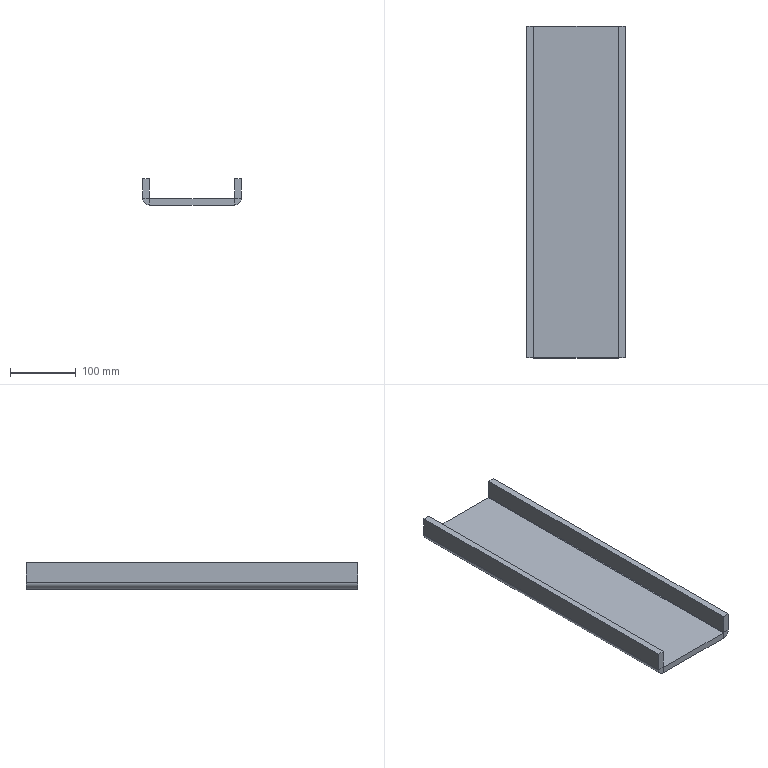Component | SolidWorks | Stiffener,RearConnection-1 | 1 solid | 22 faces | box 150 x 506 x 40 mm | volume 1037683 mm3 | plane 18 | cylinder 4 | commonest cylinder face diameters 21.473 x2 1.473 x2 | material Q235
STEP:
#1=COLOUR_RGB('',0.7922,0.8196,0.9333);
#2=FILL_AREA_STYLE_COLOUR('',#1);
#3=FILL_AREA_STYLE('',(#2));
#4=SURFACE_STYLE_FILL_AREA(#3);
#5=SURFACE_SIDE_STYLE('',(#4));
#6=SURFACE_STYLE_USAGE(.BOTH.,#5);
#7=PRESENTATION_STYLE_ASSIGNMENT((#6));
#8=CARTESIAN_POINT('',(-34.721,-42.659,92.429));
#9=VERTEX_POINT('',#8);
#10=CARTESIAN_POINT('',(-34.721,-22.737,92.429));
#11=VERTEX_POINT('',#10);
#12=CARTESIAN_POINT('',(-34.721,-42.659,92.429));
#13=DIRECTION('',(-0.,1.,-0.));
#14=VECTOR('',#13,39.37);
#15=LINE('',#12,#14);
#16=EDGE_CURVE('',#9,#11,#15,.T.);
#17=ORIENTED_EDGE('',*,*,#16,.T.);
#18=CARTESIAN_POINT('',(-29.661,-22.737,92.429));
#19=VERTEX_POINT('',#18);
#20=CARTESIAN_POINT('',(-29.238,-22.737,92.429));
#21=DIRECTION('',(-1.,-0.,0.));
#22=VECTOR('',#21,39.37);
#23=LINE('',#20,#22);
#24=EDGE_CURVE('',#19,#11,#23,.T.);
#25=ORIENTED_EDGE('',*,*,#24,.F.);
#26=CARTESIAN_POINT('',(-29.661,-42.659,92.429));
#27=VERTEX_POINT('',#26);
#28=CARTESIAN_POINT('',(-29.661,-22.737,92.429));
#29=DIRECTION('',(0.,-1.,0.));
#30=VECTOR('',#29,39.37);
#31=LINE('',#28,#30);
#32=EDGE_CURVE('',#19,#27,#31,.T.);
#33=ORIENTED_EDGE('',*,*,#32,.T.);
#34=CARTESIAN_POINT('',(-29.238,-42.659,92.429));
#35=DIRECTION('',(1.,0.,-0.));
#36=VECTOR('',#35,39.37);
#37=LINE('',#34,#36);
#38=EDGE_CURVE('',#9,#27,#37,.T.);
#39=ORIENTED_EDGE('',*,*,#38,.F.);
#40=EDGE_LOOP('',(#17,#25,#33,#39));
#41=FACE_OUTER_BOUND('',#40,.T.);
#42=CARTESIAN_POINT('',(-32.191,-32.698,92.429));
#43=DIRECTION('',(0.,0.,1.));
#44=DIRECTION('',(0.,-1.,0.));
#45=AXIS2_PLACEMENT_3D('',#42,#43,#44);
#46=PLANE('',#45);
#47=ADVANCED_FACE('',(#41),#46,.F.);
#48=CARTESIAN_POINT('',(-29.661,-22.737,92.823));
#49=VERTEX_POINT('',#48);
#50=CARTESIAN_POINT('',(-34.721,-22.737,92.823));
#51=VERTEX_POINT('',#50);
#52=CARTESIAN_POINT('',(-29.238,-22.737,92.823));
#53=DIRECTION('',(-1.,-0.,0.));
#54=VECTOR('',#53,39.37);
#55=LINE('',#52,#54);
#56=EDGE_CURVE('',#49,#51,#55,.T.);
#57=ORIENTED_EDGE('',*,*,#56,.T.);
#58=CARTESIAN_POINT('',(-34.721,-42.659,92.823));
#59=VERTEX_POINT('',#58);
#60=CARTESIAN_POINT('',(-34.721,-42.659,92.823));
#61=DIRECTION('',(-0.,1.,-0.));
#62=VECTOR('',#61,39.37);
#63=LINE('',#60,#62);
#64=EDGE_CURVE('',#59,#51,#63,.T.);
#65=ORIENTED_EDGE('',*,*,#64,.F.);
#66=CARTESIAN_POINT('',(-29.661,-42.659,92.823));
#67=VERTEX_POINT('',#66);
#68=CARTESIAN_POINT('',(-29.238,-42.659,92.823));
#69=DIRECTION('',(1.,0.,-0.));
#70=VECTOR('',#69,39.37);
#71=LINE('',#68,#70);
#72=EDGE_CURVE('',#59,#67,#71,.T.);
#73=ORIENTED_EDGE('',*,*,#72,.T.);
#74=CARTESIAN_POINT('',(-29.661,-22.737,92.823));
#75=DIRECTION('',(0.,-1.,0.));
#76=VECTOR('',#75,39.37);
#77=LINE('',#74,#76);
#78=EDGE_CURVE('',#49,#67,#77,.T.);
#79=ORIENTED_EDGE('',*,*,#78,.F.);
#80=EDGE_LOOP('',(#57,#65,#73,#79));
#81=FACE_OUTER_BOUND('',#80,.T.);
#82=CARTESIAN_POINT('',(-32.191,-32.698,92.823));
#83=DIRECTION('',(0.,0.,1.));
#84=DIRECTION('',(0.,-1.,0.));
#85=AXIS2_PLACEMENT_3D('',#82,#83,#84);
#86=PLANE('',#85);
#87=ADVANCED_FACE('',(#81),#86,.T.);
#88=ORIENTED_EDGE('',*,*,#72,.F.);
#89=CARTESIAN_POINT('',(-34.721,-42.659,92.823));
#90=DIRECTION('',(-0.,-0.,-1.));
#91=VECTOR('',#90,39.37);
#92=LINE('',#89,#91);
#93=EDGE_CURVE('',#59,#9,#92,.T.);
#94=ORIENTED_EDGE('',*,*,#93,.T.);
#95=ORIENTED_EDGE('',*,*,#38,.T.);
#96=CARTESIAN_POINT('',(-29.661,-42.659,92.823));
#97=DIRECTION('',(-0.,-0.,-1.));
#98=VECTOR('',#97,39.37);
#99=LINE('',#96,#98);
#100=EDGE_CURVE('',#67,#27,#99,.T.);
#101=ORIENTED_EDGE('',*,*,#100,.F.);
#102=EDGE_LOOP('',(#88,#94,#95,#101));
#103=FACE_OUTER_BOUND('',#102,.T.);
#104=CARTESIAN_POINT('',(-29.238,-42.659,92.429));
#105=DIRECTION('',(0.,-1.,0.));
#106=DIRECTION('',(-0.,-0.,-1.));
#107=AXIS2_PLACEMENT_3D('',#104,#105,#106);
#108=PLANE('',#107);
#109=ADVANCED_FACE('',(#103),#108,.T.);
#110=CARTESIAN_POINT('',(-34.721,-22.737,92.823));
#111=DIRECTION('',(-0.,-0.,-1.));
#112=VECTOR('',#111,39.37);
#113=LINE('',#110,#112);
#114=EDGE_CURVE('',#51,#11,#113,.T.);
#115=ORIENTED_EDGE('',*,*,#114,.F.);
#116=ORIENTED_EDGE('',*,*,#56,.F.);
#117=CARTESIAN_POINT('',(-29.661,-22.737,92.823));
#118=DIRECTION('',(-0.,-0.,-1.));
#119=VECTOR('',#118,39.37);
#120=LINE('',#117,#119);
#121=EDGE_CURVE('',#49,#19,#120,.T.);
#122=ORIENTED_EDGE('',*,*,#121,.T.);
#123=ORIENTED_EDGE('',*,*,#24,.T.);
#124=EDGE_LOOP('',(#115,#116,#122,#123));
#125=FACE_OUTER_BOUND('',#124,.T.);
#126=CARTESIAN_POINT('',(-29.238,-22.737,92.429));
#127=DIRECTION('',(-0.,1.,-0.));
#128=DIRECTION('',(0.,0.,1.));
#129=AXIS2_PLACEMENT_3D('',#126,#127,#128);
#130=PLANE('',#129);
#131=ADVANCED_FACE('',(#125),#130,.T.);
#132=CARTESIAN_POINT('',(-29.632,-42.659,92.852));
#133=VERTEX_POINT('',#132);
#134=CARTESIAN_POINT('',(-29.238,-42.659,92.852));
#135=VERTEX_POINT('',#134);
#136=CARTESIAN_POINT('',(-29.238,-42.659,92.852));
#137=DIRECTION('',(1.,0.,-0.));
#138=VECTOR('',#137,39.37);
#139=LINE('',#136,#138);
#140=EDGE_CURVE('',#133,#135,#139,.T.);
#141=ORIENTED_EDGE('',*,*,#140,.F.);
#142=CARTESIAN_POINT('',(-29.661,-42.659,92.852));
#143=DIRECTION('',(0.,-1.,0.));
#144=DIRECTION('',(0.,0.,1.));
#145=AXIS2_PLACEMENT_3D('',#142,#143,#144);
#146=CIRCLE('',#145,0.029);
#147=EDGE_CURVE('',#67,#133,#146,.T.);
#148=ORIENTED_EDGE('',*,*,#147,.F.);
#149=ORIENTED_EDGE('',*,*,#100,.T.);
#150=CARTESIAN_POINT('',(-29.661,-42.659,92.852));
#151=DIRECTION('',(0.,-1.,0.));
#152=DIRECTION('',(0.,0.,1.));
#153=AXIS2_PLACEMENT_3D('',#150,#151,#152);
#154=CIRCLE('',#153,0.4227);
#155=EDGE_CURVE('',#27,#135,#154,.T.);
#156=ORIENTED_EDGE('',*,*,#155,.T.);
#157=EDGE_LOOP('',(#141,#148,#149,#156));
#158=FACE_OUTER_BOUND('',#157,.T.);
#159=CARTESIAN_POINT('',(-29.661,-42.659,92.852));
#160=DIRECTION('',(0.,-1.,0.));
#161=DIRECTION('',(-0.,-0.,-1.));
#162=AXIS2_PLACEMENT_3D('',#159,#160,#161);
#163=PLANE('',#162);
#164=ADVANCED_FACE('',(#158),#163,.T.);
#165=CARTESIAN_POINT('',(-29.632,-22.737,92.852));
#166=VERTEX_POINT('',#165);
#167=CARTESIAN_POINT('',(-29.661,-22.737,92.852));
#168=DIRECTION('',(-0.,1.,-0.));
#169=DIRECTION('',(0.,0.,1.));
#170=AXIS2_PLACEMENT_3D('',#167,#168,#169);
#171=CIRCLE('',#170,0.029);
#172=EDGE_CURVE('',#166,#49,#171,.T.);
#173=ORIENTED_EDGE('',*,*,#172,.F.);
#174=CARTESIAN_POINT('',(-29.238,-22.737,92.852));
#175=VERTEX_POINT('',#174);
#176=CARTESIAN_POINT('',(-29.632,-22.737,92.852));
#177=DIRECTION('',(1.,0.,-0.));
#178=VECTOR('',#177,39.37);
#179=LINE('',#176,#178);
#180=EDGE_CURVE('',#166,#175,#179,.T.);
#181=ORIENTED_EDGE('',*,*,#180,.T.);
#182=CARTESIAN_POINT('',(-29.661,-22.737,92.852));
#183=DIRECTION('',(-0.,1.,-0.));
#184=DIRECTION('',(0.,0.,1.));
#185=AXIS2_PLACEMENT_3D('',#182,#183,#184);
#186=CIRCLE('',#185,0.4227);
#187=EDGE_CURVE('',#175,#19,#186,.T.);
#188=ORIENTED_EDGE('',*,*,#187,.T.);
#189=ORIENTED_EDGE('',*,*,#121,.F.);
#190=EDGE_LOOP('',(#173,#181,#188,#189));
#191=FACE_OUTER_BOUND('',#190,.T.);
#192=CARTESIAN_POINT('',(-29.661,-22.737,92.852));
#193=DIRECTION('',(0.,-1.,0.));
#194=DIRECTION('',(-0.,-0.,-1.));
#195=AXIS2_PLACEMENT_3D('',#192,#193,#194);
#196=PLANE('',#195);
#197=ADVANCED_FACE('',(#191),#196,.F.);
#198=ORIENTED_EDGE('',*,*,#32,.F.);
#199=ORIENTED_EDGE('',*,*,#187,.F.);
#200=CARTESIAN_POINT('',(-29.238,-32.698,92.852));
#201=DIRECTION('',(-0.,1.,-0.));
#202=VECTOR('',#201,39.37);
#203=LINE('',#200,#202);
#204=EDGE_CURVE('',#135,#175,#203,.T.);
#205=ORIENTED_EDGE('',*,*,#204,.F.);
#206=ORIENTED_EDGE('',*,*,#155,.F.);
#207=EDGE_LOOP('',(#198,#199,#205,#206));
#208=FACE_OUTER_BOUND('',#207,.T.);
#209=CARTESIAN_POINT('',(-29.661,-22.737,92.852));
#210=DIRECTION('',(-0.,1.,-0.));
#211=DIRECTION('',(1.,0.,0.));
#212=AXIS2_PLACEMENT_3D('',#209,#210,#211);
#213=CYLINDRICAL_SURFACE('',#212,0.4227);
#214=ADVANCED_FACE('',(#208),#213,.T.);
#215=ORIENTED_EDGE('',*,*,#78,.T.);
#216=ORIENTED_EDGE('',*,*,#147,.T.);
#217=CARTESIAN_POINT('',(-29.632,-42.659,92.852));
#218=DIRECTION('',(-0.,1.,-0.));
#219=VECTOR('',#218,39.37);
#220=LINE('',#217,#219);
#221=EDGE_CURVE('',#133,#166,#220,.T.);
#222=ORIENTED_EDGE('',*,*,#221,.T.);
#223=ORIENTED_EDGE('',*,*,#172,.T.);
#224=EDGE_LOOP('',(#215,#216,#222,#223));
#225=FACE_OUTER_BOUND('',#224,.T.);
#226=CARTESIAN_POINT('',(-29.661,-22.737,92.852));
#227=DIRECTION('',(-0.,1.,-0.));
#228=DIRECTION('',(1.,0.,0.));
#229=AXIS2_PLACEMENT_3D('',#226,#227,#228);
#230=CYLINDRICAL_SURFACE('',#229,0.029);
#231=ADVANCED_FACE('',(#225),#230,.F.);
#232=CARTESIAN_POINT('',(-29.238,-22.737,94.004));
#233=VERTEX_POINT('',#232);
#234=CARTESIAN_POINT('',(-29.238,-22.737,92.823));
#235=DIRECTION('',(-0.,-0.,-1.));
#236=VECTOR('',#235,39.37);
#237=LINE('',#234,#236);
#238=EDGE_CURVE('',#233,#175,#237,.T.);
#239=ORIENTED_EDGE('',*,*,#238,.T.);
#240=ORIENTED_EDGE('',*,*,#180,.F.);
#241=CARTESIAN_POINT('',(-29.632,-22.737,94.004));
#242=VERTEX_POINT('',#241);
#243=CARTESIAN_POINT('',(-29.632,-22.737,92.823));
#244=DIRECTION('',(-0.,-0.,-1.));
#245=VECTOR('',#244,39.37);
#246=LINE('',#243,#245);
#247=EDGE_CURVE('',#242,#166,#246,.T.);
#248=ORIENTED_EDGE('',*,*,#247,.F.);
#249=CARTESIAN_POINT('',(-29.238,-22.737,94.004));
#250=DIRECTION('',(-1.,-0.,0.));
#251=VECTOR('',#250,39.37);
#252=LINE('',#249,#251);
#253=EDGE_CURVE('',#233,#242,#252,.T.);
#254=ORIENTED_EDGE('',*,*,#253,.F.);
#255=EDGE_LOOP('',(#239,#240,#248,#254));
#256=FACE_OUTER_BOUND('',#255,.T.);
#257=CARTESIAN_POINT('',(-29.238,-22.737,92.823));
#258=DIRECTION('',(-0.,1.,-0.));
#259=DIRECTION('',(0.,0.,1.));
#260=AXIS2_PLACEMENT_3D('',#257,#258,#259);
#261=PLANE('',#260);
#262=ADVANCED_FACE('',(#256),#261,.T.);
#263=CARTESIAN_POINT('',(-29.632,-42.659,94.004));
#264=VERTEX_POINT('',#263);
#265=CARTESIAN_POINT('',(-29.632,-42.659,92.823));
#266=DIRECTION('',(0.,0.,1.));
#267=VECTOR('',#266,39.37);
#268=LINE('',#265,#267);
#269=EDGE_CURVE('',#133,#264,#268,.T.);
#270=ORIENTED_EDGE('',*,*,#269,.F.);
#271=ORIENTED_EDGE('',*,*,#140,.T.);
#272=CARTESIAN_POINT('',(-29.238,-42.659,94.004));
#273=VERTEX_POINT('',#272);
#274=CARTESIAN_POINT('',(-29.238,-42.659,94.004));
#275=DIRECTION('',(0.,0.,1.));
#276=VECTOR('',#275,39.37);
#277=LINE('',#274,#276);
#278=EDGE_CURVE('',#135,#273,#277,.T.);
#279=ORIENTED_EDGE('',*,*,#278,.T.);
#280=CARTESIAN_POINT('',(-29.238,-42.659,94.004));
#281=DIRECTION('',(-1.,-0.,0.));
#282=VECTOR('',#281,39.37);
#283=LINE('',#280,#282);
#284=EDGE_CURVE('',#273,#264,#283,.T.);
#285=ORIENTED_EDGE('',*,*,#284,.T.);
#286=EDGE_LOOP('',(#270,#271,#279,#285));
#287=FACE_OUTER_BOUND('',#286,.T.);
#288=CARTESIAN_POINT('',(-29.238,-42.659,94.004));
#289=DIRECTION('',(0.,-1.,0.));
#290=DIRECTION('',(-0.,-0.,-1.));
#291=AXIS2_PLACEMENT_3D('',#288,#289,#290);
#292=PLANE('',#291);
#293=ADVANCED_FACE('',(#287),#292,.T.);
#294=ORIENTED_EDGE('',*,*,#278,.F.);
#295=ORIENTED_EDGE('',*,*,#204,.T.);
#296=ORIENTED_EDGE('',*,*,#238,.F.);
#297=CARTESIAN_POINT('',(-29.238,-22.737,94.004));
#298=DIRECTION('',(-0.,1.,-0.));
#299=VECTOR('',#298,39.37);
#300=LINE('',#297,#299);
#301=EDGE_CURVE('',#273,#233,#300,.T.);
#302=ORIENTED_EDGE('',*,*,#301,.F.);
#303=EDGE_LOOP('',(#294,#295,#296,#302));
#304=FACE_OUTER_BOUND('',#303,.T.);
#305=CARTESIAN_POINT('',(-29.238,-32.698,92.823));
#306=DIRECTION('',(1.,0.,-0.));
#307=DIRECTION('',(0.,0.,1.));
#308=AXIS2_PLACEMENT_3D('',#305,#306,#307);
#309=PLANE('',#308);
#310=ADVANCED_FACE('',(#304),#309,.T.);
#311=ORIENTED_EDGE('',*,*,#221,.F.);
#312=ORIENTED_EDGE('',*,*,#269,.T.);
#313=CARTESIAN_POINT('',(-29.632,-32.698,94.004));
#314=DIRECTION('',(-0.,1.,-0.));
#315=VECTOR('',#314,39.37);
#316=LINE('',#313,#315);
#317=EDGE_CURVE('',#264,#242,#316,.T.);
#318=ORIENTED_EDGE('',*,*,#317,.T.);
#319=ORIENTED_EDGE('',*,*,#247,.T.);
#320=EDGE_LOOP('',(#311,#312,#318,#319));
#321=FACE_OUTER_BOUND('',#320,.T.);
#322=CARTESIAN_POINT('',(-29.632,-32.698,92.823));
#323=DIRECTION('',(1.,0.,-0.));
#324=DIRECTION('',(0.,0.,1.));
#325=AXIS2_PLACEMENT_3D('',#322,#323,#324);
#326=PLANE('',#325);
#327=ADVANCED_FACE('',(#321),#326,.F.);
#328=ORIENTED_EDGE('',*,*,#317,.F.);
#329=ORIENTED_EDGE('',*,*,#284,.F.);
#330=ORIENTED_EDGE('',*,*,#301,.T.);
#331=ORIENTED_EDGE('',*,*,#253,.T.);
#332=EDGE_LOOP('',(#328,#329,#330,#331));
#333=FACE_OUTER_BOUND('',#332,.T.);
#334=CARTESIAN_POINT('',(-29.238,-22.737,94.004));
#335=DIRECTION('',(0.,0.,1.));
#336=DIRECTION('',(-1.,-0.,0.));
#337=AXIS2_PLACEMENT_3D('',#334,#335,#336);
#338=PLANE('',#337);
#339=ADVANCED_FACE('',(#333),#338,.T.);
#340=CARTESIAN_POINT('',(-34.75,-22.737,92.852));
#341=VERTEX_POINT('',#340);
#342=CARTESIAN_POINT('',(-35.144,-22.737,92.852));
#343=VERTEX_POINT('',#342);
#344=CARTESIAN_POINT('',(-35.144,-22.737,92.852));
#345=DIRECTION('',(-1.,-0.,0.));
#346=VECTOR('',#345,39.37);
#347=LINE('',#344,#346);
#348=EDGE_CURVE('',#341,#343,#347,.T.);
#349=ORIENTED_EDGE('',*,*,#348,.F.);
#350=CARTESIAN_POINT('',(-34.721,-22.737,92.852));
#351=DIRECTION('',(-0.,1.,-0.));
#352=DIRECTION('',(0.,0.,-1.));
#353=AXIS2_PLACEMENT_3D('',#350,#351,#352);
#354=CIRCLE('',#353,0.029);
#355=EDGE_CURVE('',#51,#341,#354,.T.);
#356=ORIENTED_EDGE('',*,*,#355,.F.);
#357=ORIENTED_EDGE('',*,*,#114,.T.);
#358=CARTESIAN_POINT('',(-34.721,-22.737,92.852));
#359=DIRECTION('',(-0.,1.,-0.));
#360=DIRECTION('',(-0.,0.,-1.));
#361=AXIS2_PLACEMENT_3D('',#358,#359,#360);
#362=CIRCLE('',#361,0.4227);
#363=EDGE_CURVE('',#11,#343,#362,.T.);
#364=ORIENTED_EDGE('',*,*,#363,.T.);
#365=EDGE_LOOP('',(#349,#356,#357,#364));
#366=FACE_OUTER_BOUND('',#365,.T.);
#367=CARTESIAN_POINT('',(-34.721,-22.737,92.852));
#368=DIRECTION('',(-0.,1.,-0.));
#369=DIRECTION('',(0.,0.,1.));
#370=AXIS2_PLACEMENT_3D('',#367,#368,#369);
#371=PLANE('',#370);
#372=ADVANCED_FACE('',(#366),#371,.T.);
#373=CARTESIAN_POINT('',(-34.75,-42.659,92.852));
#374=VERTEX_POINT('',#373);
#375=CARTESIAN_POINT('',(-34.721,-42.659,92.852));
#376=DIRECTION('',(0.,-1.,0.));
#377=DIRECTION('',(0.,0.,-1.));
#378=AXIS2_PLACEMENT_3D('',#375,#376,#377);
#379=CIRCLE('',#378,0.029);
#380=EDGE_CURVE('',#374,#59,#379,.T.);
#381=ORIENTED_EDGE('',*,*,#380,.F.);
#382=CARTESIAN_POINT('',(-35.144,-42.659,92.852));
#383=VERTEX_POINT('',#382);
#384=CARTESIAN_POINT('',(-34.75,-42.659,92.852));
#385=DIRECTION('',(-1.,-0.,0.));
#386=VECTOR('',#385,39.37);
#387=LINE('',#384,#386);
#388=EDGE_CURVE('',#374,#383,#387,.T.);
#389=ORIENTED_EDGE('',*,*,#388,.T.);
#390=CARTESIAN_POINT('',(-34.721,-42.659,92.852));
#391=DIRECTION('',(0.,-1.,0.));
#392=DIRECTION('',(0.,0.,-1.));
#393=AXIS2_PLACEMENT_3D('',#390,#391,#392);
#394=CIRCLE('',#393,0.4227);
#395=EDGE_CURVE('',#383,#9,#394,.T.);
#396=ORIENTED_EDGE('',*,*,#395,.T.);
#397=ORIENTED_EDGE('',*,*,#93,.F.);
#398=EDGE_LOOP('',(#381,#389,#396,#397));
#399=FACE_OUTER_BOUND('',#398,.T.);
#400=CARTESIAN_POINT('',(-34.721,-42.659,92.852));
#401=DIRECTION('',(-0.,1.,-0.));
#402=DIRECTION('',(0.,0.,1.));
#403=AXIS2_PLACEMENT_3D('',#400,#401,#402);
#404=PLANE('',#403);
#405=ADVANCED_FACE('',(#399),#404,.F.);
#406=ORIENTED_EDGE('',*,*,#16,.F.);
#407=ORIENTED_EDGE('',*,*,#395,.F.);
#408=CARTESIAN_POINT('',(-35.144,-32.698,92.852));
#409=DIRECTION('',(0.,-1.,0.));
#410=VECTOR('',#409,39.37);
#411=LINE('',#408,#410);
#412=EDGE_CURVE('',#343,#383,#411,.T.);
#413=ORIENTED_EDGE('',*,*,#412,.F.);
#414=ORIENTED_EDGE('',*,*,#363,.F.);
#415=EDGE_LOOP('',(#406,#407,#413,#414));
#416=FACE_OUTER_BOUND('',#415,.T.);
#417=CARTESIAN_POINT('',(-34.721,-42.659,92.852));
#418=DIRECTION('',(0.,-1.,0.));
#419=DIRECTION('',(-1.,0.,0.));
#420=AXIS2_PLACEMENT_3D('',#417,#418,#419);
#421=CYLINDRICAL_SURFACE('',#420,0.4227);
#422=ADVANCED_FACE('',(#416),#421,.T.);
#423=ORIENTED_EDGE('',*,*,#64,.T.);
#424=ORIENTED_EDGE('',*,*,#355,.T.);
#425=CARTESIAN_POINT('',(-34.75,-22.737,92.852));
#426=DIRECTION('',(0.,-1.,0.));
#427=VECTOR('',#426,39.37);
#428=LINE('',#425,#427);
#429=EDGE_CURVE('',#341,#374,#428,.T.);
#430=ORIENTED_EDGE('',*,*,#429,.T.);
#431=ORIENTED_EDGE('',*,*,#380,.T.);
#432=EDGE_LOOP('',(#423,#424,#430,#431));
#433=FACE_OUTER_BOUND('',#432,.T.);
#434=CARTESIAN_POINT('',(-34.721,-42.659,92.852));
#435=DIRECTION('',(0.,-1.,0.));
#436=DIRECTION('',(-1.,0.,0.));
#437=AXIS2_PLACEMENT_3D('',#434,#435,#436);
#438=CYLINDRICAL_SURFACE('',#437,0.029);
#439=ADVANCED_FACE('',(#433),#438,.F.);
#440=CARTESIAN_POINT('',(-35.144,-42.659,94.004));
#441=VERTEX_POINT('',#440);
#442=CARTESIAN_POINT('',(-35.144,-42.659,92.823));
#443=DIRECTION('',(-0.,-0.,-1.));
#444=VECTOR('',#443,39.37);
#445=LINE('',#442,#444);
#446=EDGE_CURVE('',#441,#383,#445,.T.);
#447=ORIENTED_EDGE('',*,*,#446,.T.);
#448=ORIENTED_EDGE('',*,*,#388,.F.);
#449=CARTESIAN_POINT('',(-34.75,-42.659,94.004));
#450=VERTEX_POINT('',#449);
#451=CARTESIAN_POINT('',(-34.75,-42.659,92.823));
#452=DIRECTION('',(-0.,-0.,-1.));
#453=VECTOR('',#452,39.37);
#454=LINE('',#451,#453);
#455=EDGE_CURVE('',#450,#374,#454,.T.);
#456=ORIENTED_EDGE('',*,*,#455,.F.);
#457=CARTESIAN_POINT('',(-35.144,-42.659,94.004));
#458=DIRECTION('',(1.,0.,-0.));
#459=VECTOR('',#458,39.37);
#460=LINE('',#457,#459);
#461=EDGE_CURVE('',#441,#450,#460,.T.);
#462=ORIENTED_EDGE('',*,*,#461,.F.);
#463=EDGE_LOOP('',(#447,#448,#456,#462));
#464=FACE_OUTER_BOUND('',#463,.T.);
#465=CARTESIAN_POINT('',(-35.144,-42.659,92.823));
#466=DIRECTION('',(0.,-1.,0.));
#467=DIRECTION('',(-0.,-0.,-1.));
#468=AXIS2_PLACEMENT_3D('',#465,#466,#467);
#469=PLANE('',#468);
#470=ADVANCED_FACE('',(#464),#469,.T.);
#471=CARTESIAN_POINT('',(-34.75,-22.737,94.004));
#472=VERTEX_POINT('',#471);
#473=CARTESIAN_POINT('',(-34.75,-22.737,92.823));
#474=DIRECTION('',(0.,0.,1.));
#475=VECTOR('',#474,39.37);
#476=LINE('',#473,#475);
#477=EDGE_CURVE('',#341,#472,#476,.T.);
#478=ORIENTED_EDGE('',*,*,#477,.F.);
#479=ORIENTED_EDGE('',*,*,#348,.T.);
#480=CARTESIAN_POINT('',(-35.144,-22.737,94.004));
#481=VERTEX_POINT('',#480);
#482=CARTESIAN_POINT('',(-35.144,-22.737,94.004));
#483=DIRECTION('',(0.,0.,1.));
#484=VECTOR('',#483,39.37);
#485=LINE('',#482,#484);
#486=EDGE_CURVE('',#343,#481,#485,.T.);
#487=ORIENTED_EDGE('',*,*,#486,.T.);
#488=CARTESIAN_POINT('',(-35.144,-22.737,94.004));
#489=DIRECTION('',(1.,0.,-0.));
#490=VECTOR('',#489,39.37);
#491=LINE('',#488,#490);
#492=EDGE_CURVE('',#481,#472,#491,.T.);
#493=ORIENTED_EDGE('',*,*,#492,.T.);
#494=EDGE_LOOP('',(#478,#479,#487,#493));
#495=FACE_OUTER_BOUND('',#494,.T.);
#496=CARTESIAN_POINT('',(-35.144,-22.737,94.004));
#497=DIRECTION('',(-0.,1.,-0.));
#498=DIRECTION('',(0.,0.,1.));
#499=AXIS2_PLACEMENT_3D('',#496,#497,#498);
#500=PLANE('',#499);
#501=ADVANCED_FACE('',(#495),#500,.T.);
#502=ORIENTED_EDGE('',*,*,#486,.F.);
#503=ORIENTED_EDGE('',*,*,#412,.T.);
#504=ORIENTED_EDGE('',*,*,#446,.F.);
#505=CARTESIAN_POINT('',(-35.144,-42.659,94.004));
#506=DIRECTION('',(0.,-1.,0.));
#507=VECTOR('',#506,39.37);
#508=LINE('',#505,#507);
#509=EDGE_CURVE('',#481,#441,#508,.T.);
#510=ORIENTED_EDGE('',*,*,#509,.F.);
#511=EDGE_LOOP('',(#502,#503,#504,#510));
#512=FACE_OUTER_BOUND('',#511,.T.);
#513=CARTESIAN_POINT('',(-35.144,-32.698,92.823));
#514=DIRECTION('',(-1.,-0.,0.));
#515=DIRECTION('',(-0.,-0.,-1.));
#516=AXIS2_PLACEMENT_3D('',#513,#514,#515);
#517=PLANE('',#516);
#518=ADVANCED_FACE('',(#512),#517,.T.);
#519=ORIENTED_EDGE('',*,*,#429,.F.);
#520=ORIENTED_EDGE('',*,*,#477,.T.);
#521=CARTESIAN_POINT('',(-34.75,-32.698,94.004));
#522=DIRECTION('',(0.,-1.,0.));
#523=VECTOR('',#522,39.37);
#524=LINE('',#521,#523);
#525=EDGE_CURVE('',#472,#450,#524,.T.);
#526=ORIENTED_EDGE('',*,*,#525,.T.);
#527=ORIENTED_EDGE('',*,*,#455,.T.);
#528=EDGE_LOOP('',(#519,#520,#526,#527));
#529=FACE_OUTER_BOUND('',#528,.T.);
#530=CARTESIAN_POINT('',(-34.75,-32.698,92.823));
#531=DIRECTION('',(-1.,-0.,0.));
#532=DIRECTION('',(-0.,-0.,-1.));
#533=AXIS2_PLACEMENT_3D('',#530,#531,#532);
#534=PLANE('',#533);
#535=ADVANCED_FACE('',(#529),#534,.F.);
#536=ORIENTED_EDGE('',*,*,#525,.F.);
#537=ORIENTED_EDGE('',*,*,#492,.F.);
#538=ORIENTED_EDGE('',*,*,#509,.T.);
#539=ORIENTED_EDGE('',*,*,#461,.T.);
#540=EDGE_LOOP('',(#536,#537,#538,#539));
#541=FACE_OUTER_BOUND('',#540,.T.);
#542=CARTESIAN_POINT('',(-35.144,-42.659,94.004));
#543=DIRECTION('',(0.,0.,1.));
#544=DIRECTION('',(-1.,-0.,0.));
#545=AXIS2_PLACEMENT_3D('',#542,#543,#544);
#546=PLANE('',#545);
#547=ADVANCED_FACE('',(#541),#546,.T.);
#548=CLOSED_SHELL('',(#47,#87,#109,#131,#164,#197,#214,#231,#262,#293,#310,#327,#339,#372,#405,#422,#439,#470,#501,#518,#535,#547));
#549=MANIFOLD_SOLID_BREP('',#548);
#550=STYLED_ITEM('',(#7),#549);
#551=PRESENTATION_LAYER_ASSIGNMENT('','',(#550));
#552=CARTESIAN_POINT('',(0.,0.,0.));
#553=DIRECTION('',(0.,0.,1.));
#554=DIRECTION('',(1.,0.,0.));
#555=AXIS2_PLACEMENT_3D('',#552,#553,#554);
#556=(LENGTH_UNIT()NAMED_UNIT(*)SI_UNIT($,.METRE.));
#557=LENGTH_MEASURE_WITH_UNIT(LENGTH_MEASURE(0.0254),#556);
#558=DIMENSIONAL_EXPONENTS(1.,0.,0.,0.,0.,0.,0.);
#559=(CONVERSION_BASED_UNIT('',#557)LENGTH_UNIT()NAMED_UNIT(#558));
#560=UNCERTAINTY_MEASURE_WITH_UNIT(LENGTH_MEASURE(0.00001),#559,'','');
#561=(NAMED_UNIT(*)PLANE_ANGLE_UNIT()SI_UNIT($,.RADIAN.));
#562=(NAMED_UNIT(*)SI_UNIT($,.STERADIAN.)SOLID_ANGLE_UNIT());
#563=(GEOMETRIC_REPRESENTATION_CONTEXT(3)GLOBAL_UNCERTAINTY_ASSIGNED_CONTEXT((#560))GLOBAL_UNIT_ASSIGNED_CONTEXT((#559,#561,#562))REPRESENTATION_CONTEXT('',''));
#564=ADVANCED_BREP_SHAPE_REPRESENTATION('',(#549,#555),#563);
#565=(LENGTH_UNIT()NAMED_UNIT(*)SI_UNIT($,.METRE.));
#566=LENGTH_MEASURE_WITH_UNIT(LENGTH_MEASURE(0.0254),#565);
#567=DIMENSIONAL_EXPONENTS(1.,0.,0.,0.,0.,0.,0.);
#568=(CONVERSION_BASED_UNIT('',#566)LENGTH_UNIT()NAMED_UNIT(#567));
#569=UNCERTAINTY_MEASURE_WITH_UNIT(LENGTH_MEASURE(0.00001),#568,'','');
#570=(NAMED_UNIT(*)PLANE_ANGLE_UNIT()SI_UNIT($,.RADIAN.));
#571=(NAMED_UNIT(*)SI_UNIT($,.STERADIAN.)SOLID_ANGLE_UNIT());
#572=(GEOMETRIC_REPRESENTATION_CONTEXT(3)GLOBAL_UNCERTAINTY_ASSIGNED_CONTEXT((#569))GLOBAL_UNIT_ASSIGNED_CONTEXT((#568,#570,#571))REPRESENTATION_CONTEXT('',''));
#573=MECHANICAL_DESIGN_GEOMETRIC_PRESENTATION_REPRESENTATION('',(#550),#572);